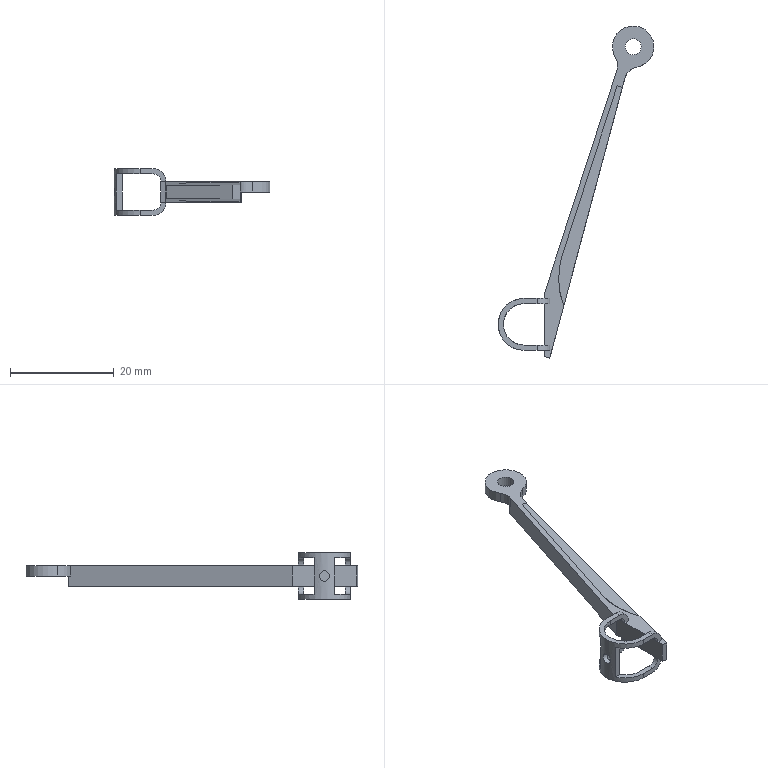Component | NX | 05 | 1 solid | 53 faces | volume 442 mm3 | plane 36 | cylinder 17 | commonest cylinder face diameters 5 x4 3 x4 6 x2 30 x2 8 x2 3.1 x1 10 x1 2 x1